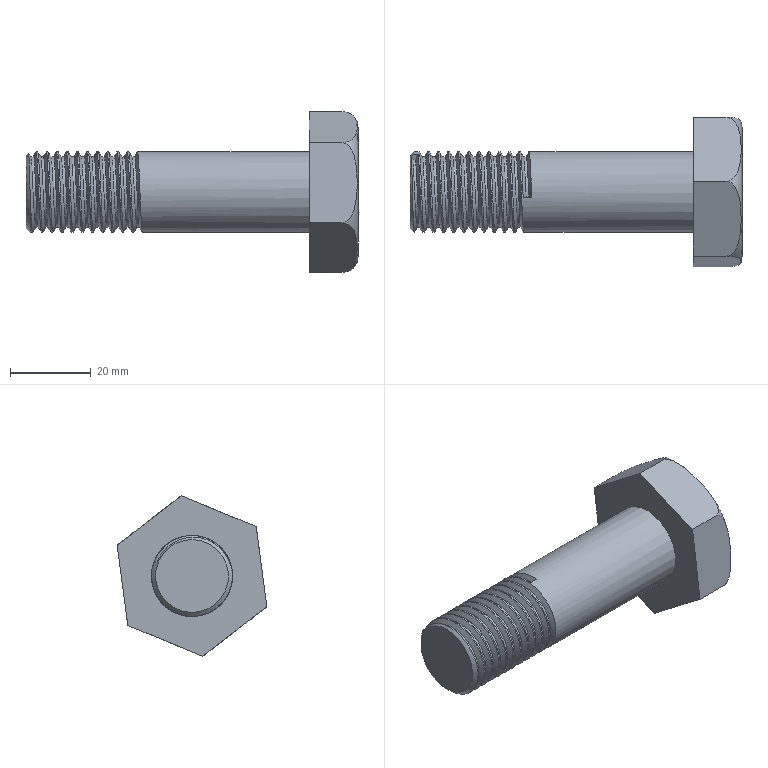Component | NX | CCJ-013 | 2 solids | 29 faces | volume 33021 mm3 | cylinder 13 | plane 12 | spline 2 | torus 1 | cone 1 | commonest cylinder face diameters 20 x12 17.5 x1